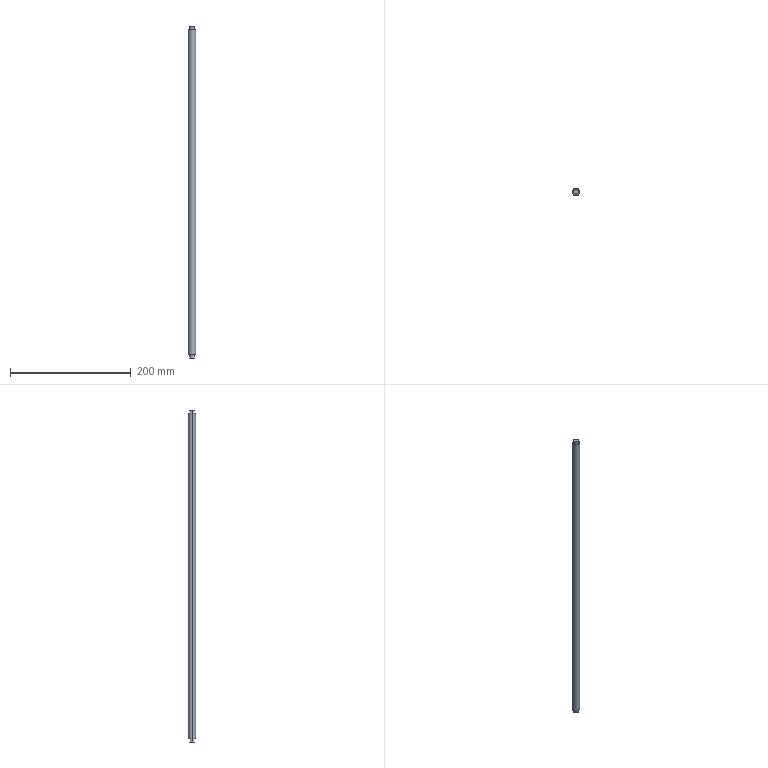Component | SolidWorks | ORTA M_L-2 | 1 solid | 10 faces | box 12 x 12 x 550 mm | volume 61575 mm3 | cylinder 6 | plane 4 | commonest cylinder face diameters 8 x4 12 x2
build123d program:
from build123d import *

# Parameters (mm, degrees)
IZIM1_R                     = 6
Y_KSEKLIK_EKSTR_ZYON1_DEPTH = 540
IZIM2_R                     = 4
Y_KSEKLIK_EKSTR_ZYON2_DEPTH = 5
Y_KSEKLIK_EKSTR_ZYON3_START = 5
IZIM3_R                     = 4
Y_KSEKLIK_EKSTR_ZYON3_DEPTH = 5


with BuildPart() as part:
    # izim1 → Y_kseklik-Ekstr_zyon1 (new body)
    with BuildSketch(Plane.XY):
        Circle(IZIM1_R)
    extrude(amount=Y_KSEKLIK_EKSTR_ZYON1_DEPTH)

    # izim2 → Y_kseklik-Ekstr_zyon2 (add)
    with BuildSketch(Plane.XY.offset(540)):
        Circle(IZIM2_R)
    extrude(amount=Y_KSEKLIK_EKSTR_ZYON2_DEPTH)

    # izim3 → Y_kseklik-Ekstr_zyon3 (add)
    with BuildSketch(Plane(origin=(0, 0, 0), x_dir=(-1, 0, 0), z_dir=(0, 0, -1)).offset(Y_KSEKLIK_EKSTR_ZYON3_START)):
        with Locations(Location((0, 0, 0), (0, 0, 180))):
            Circle(IZIM3_R)
    extrude(amount=-Y_KSEKLIK_EKSTR_ZYON3_DEPTH)


solid = part.part

# Placed as in the assembly
solid = solid.moved(Location((228.852, 24.677, -357.526), (0, 0, 0)))
STEP:
#1=COLOUR_RGB('',0.7922,0.8196,0.9333);
#2=FILL_AREA_STYLE_COLOUR('',#1);
#3=FILL_AREA_STYLE('',(#2));
#4=SURFACE_STYLE_FILL_AREA(#3);
#5=SURFACE_SIDE_STYLE('',(#4));
#6=SURFACE_STYLE_USAGE(.BOTH.,#5);
#7=PRESENTATION_STYLE_ASSIGNMENT((#6));
#8=CARTESIAN_POINT('',(8.852,0.9715,-14.273));
#9=VERTEX_POINT('',#8);
#10=CARTESIAN_POINT('',(9.167,0.9715,-14.273));
#11=VERTEX_POINT('',#10);
#12=CARTESIAN_POINT('',(9.01,0.9715,-14.273));
#13=DIRECTION('',(0.,0.,-1.));
#14=DIRECTION('',(-1.,0.,0.));
#15=AXIS2_PLACEMENT_3D('',#12,#13,#14);
#16=CIRCLE('',#15,0.1575);
#17=EDGE_CURVE('',#9,#11,#16,.T.);
#18=ORIENTED_EDGE('',*,*,#17,.F.);
#19=CARTESIAN_POINT('',(8.852,0.9715,-14.076));
#20=VERTEX_POINT('',#19);
#21=CARTESIAN_POINT('',(8.852,0.9715,-14.273));
#22=DIRECTION('',(0.,0.,1.));
#23=VECTOR('',#22,39.37);
#24=LINE('',#21,#23);
#25=EDGE_CURVE('',#9,#20,#24,.T.);
#26=ORIENTED_EDGE('',*,*,#25,.T.);
#27=CARTESIAN_POINT('',(9.167,0.9715,-14.076));
#28=VERTEX_POINT('',#27);
#29=CARTESIAN_POINT('',(9.01,0.9715,-14.076));
#30=DIRECTION('',(0.,0.,-1.));
#31=DIRECTION('',(-1.,0.,0.));
#32=AXIS2_PLACEMENT_3D('',#29,#30,#31);
#33=CIRCLE('',#32,0.1575);
#34=EDGE_CURVE('',#20,#28,#33,.T.);
#35=ORIENTED_EDGE('',*,*,#34,.T.);
#36=CARTESIAN_POINT('',(9.167,0.9715,-14.273));
#37=DIRECTION('',(0.,0.,1.));
#38=VECTOR('',#37,39.37);
#39=LINE('',#36,#38);
#40=EDGE_CURVE('',#11,#28,#39,.T.);
#41=ORIENTED_EDGE('',*,*,#40,.F.);
#42=EDGE_LOOP('',(#18,#26,#35,#41));
#43=FACE_OUTER_BOUND('',#42,.T.);
#44=CARTESIAN_POINT('',(9.01,0.9715,-14.273));
#45=DIRECTION('',(0.,0.,1.));
#46=DIRECTION('',(1.,0.,0.));
#47=AXIS2_PLACEMENT_3D('',#44,#45,#46);
#48=CYLINDRICAL_SURFACE('',#47,0.1575);
#49=ADVANCED_FACE('',(#43),#48,.T.);
#50=CARTESIAN_POINT('',(9.167,0.9715,7.381));
#51=VERTEX_POINT('',#50);
#52=CARTESIAN_POINT('',(8.852,0.9715,7.381));
#53=VERTEX_POINT('',#52);
#54=CARTESIAN_POINT('',(9.01,0.9715,7.381));
#55=DIRECTION('',(0.,0.,1.));
#56=DIRECTION('',(1.,0.,0.));
#57=AXIS2_PLACEMENT_3D('',#54,#55,#56);
#58=CIRCLE('',#57,0.1575);
#59=EDGE_CURVE('',#51,#53,#58,.T.);
#60=ORIENTED_EDGE('',*,*,#59,.F.);
#61=CARTESIAN_POINT('',(9.167,0.9715,7.184));
#62=VERTEX_POINT('',#61);
#63=CARTESIAN_POINT('',(9.167,0.9715,7.381));
#64=DIRECTION('',(0.,0.,-1.));
#65=VECTOR('',#64,39.37);
#66=LINE('',#63,#65);
#67=EDGE_CURVE('',#51,#62,#66,.T.);
#68=ORIENTED_EDGE('',*,*,#67,.T.);
#69=CARTESIAN_POINT('',(8.852,0.9715,7.184));
#70=VERTEX_POINT('',#69);
#71=CARTESIAN_POINT('',(9.01,0.9715,7.184));
#72=DIRECTION('',(0.,0.,1.));
#73=DIRECTION('',(1.,0.,0.));
#74=AXIS2_PLACEMENT_3D('',#71,#72,#73);
#75=CIRCLE('',#74,0.1575);
#76=EDGE_CURVE('',#62,#70,#75,.T.);
#77=ORIENTED_EDGE('',*,*,#76,.T.);
#78=CARTESIAN_POINT('',(8.852,0.9715,7.381));
#79=DIRECTION('',(0.,0.,-1.));
#80=VECTOR('',#79,39.37);
#81=LINE('',#78,#80);
#82=EDGE_CURVE('',#53,#70,#81,.T.);
#83=ORIENTED_EDGE('',*,*,#82,.F.);
#84=EDGE_LOOP('',(#60,#68,#77,#83));
#85=FACE_OUTER_BOUND('',#84,.T.);
#86=CARTESIAN_POINT('',(9.01,0.9715,7.381));
#87=DIRECTION('',(0.,0.,-1.));
#88=DIRECTION('',(-1.,0.,0.));
#89=AXIS2_PLACEMENT_3D('',#86,#87,#88);
#90=CYLINDRICAL_SURFACE('',#89,0.1575);
#91=ADVANCED_FACE('',(#85),#90,.T.);
#92=CARTESIAN_POINT('',(9.246,0.9715,7.184));
#93=VERTEX_POINT('',#92);
#94=CARTESIAN_POINT('',(8.774,0.9715,7.184));
#95=VERTEX_POINT('',#94);
#96=CARTESIAN_POINT('',(9.01,0.9715,7.184));
#97=DIRECTION('',(0.,0.,1.));
#98=DIRECTION('',(1.,0.,0.));
#99=AXIS2_PLACEMENT_3D('',#96,#97,#98);
#100=CIRCLE('',#99,0.2362);
#101=EDGE_CURVE('',#93,#95,#100,.T.);
#102=ORIENTED_EDGE('',*,*,#101,.F.);
#103=CARTESIAN_POINT('',(9.246,0.9715,-14.076));
#104=VERTEX_POINT('',#103);
#105=CARTESIAN_POINT('',(9.246,0.9715,7.184));
#106=DIRECTION('',(0.,0.,-1.));
#107=VECTOR('',#106,39.37);
#108=LINE('',#105,#107);
#109=EDGE_CURVE('',#93,#104,#108,.T.);
#110=ORIENTED_EDGE('',*,*,#109,.T.);
#111=CARTESIAN_POINT('',(8.774,0.9715,-14.076));
#112=VERTEX_POINT('',#111);
#113=CARTESIAN_POINT('',(9.01,0.9715,-14.076));
#114=DIRECTION('',(0.,0.,1.));
#115=DIRECTION('',(1.,0.,0.));
#116=AXIS2_PLACEMENT_3D('',#113,#114,#115);
#117=CIRCLE('',#116,0.2362);
#118=EDGE_CURVE('',#104,#112,#117,.T.);
#119=ORIENTED_EDGE('',*,*,#118,.T.);
#120=CARTESIAN_POINT('',(8.774,0.9715,7.184));
#121=DIRECTION('',(0.,0.,-1.));
#122=VECTOR('',#121,39.37);
#123=LINE('',#120,#122);
#124=EDGE_CURVE('',#95,#112,#123,.T.);
#125=ORIENTED_EDGE('',*,*,#124,.F.);
#126=EDGE_LOOP('',(#102,#110,#119,#125));
#127=FACE_OUTER_BOUND('',#126,.T.);
#128=CARTESIAN_POINT('',(9.01,0.9715,7.184));
#129=DIRECTION('',(0.,0.,-1.));
#130=DIRECTION('',(-1.,0.,0.));
#131=AXIS2_PLACEMENT_3D('',#128,#129,#130);
#132=CYLINDRICAL_SURFACE('',#131,0.2362);
#133=ADVANCED_FACE('',(#127),#132,.T.);
#134=ORIENTED_EDGE('',*,*,#109,.F.);
#135=CARTESIAN_POINT('',(9.01,0.9715,7.184));
#136=DIRECTION('',(0.,0.,1.));
#137=DIRECTION('',(1.,0.,0.));
#138=AXIS2_PLACEMENT_3D('',#135,#136,#137);
#139=CIRCLE('',#138,0.2362);
#140=EDGE_CURVE('',#95,#93,#139,.T.);
#141=ORIENTED_EDGE('',*,*,#140,.F.);
#142=ORIENTED_EDGE('',*,*,#124,.T.);
#143=CARTESIAN_POINT('',(9.01,0.9715,-14.076));
#144=DIRECTION('',(0.,0.,1.));
#145=DIRECTION('',(1.,0.,0.));
#146=AXIS2_PLACEMENT_3D('',#143,#144,#145);
#147=CIRCLE('',#146,0.2362);
#148=EDGE_CURVE('',#112,#104,#147,.T.);
#149=ORIENTED_EDGE('',*,*,#148,.T.);
#150=EDGE_LOOP('',(#134,#141,#142,#149));
#151=FACE_OUTER_BOUND('',#150,.T.);
#152=CARTESIAN_POINT('',(9.01,0.9715,7.184));
#153=DIRECTION('',(0.,0.,-1.));
#154=DIRECTION('',(-1.,0.,0.));
#155=AXIS2_PLACEMENT_3D('',#152,#153,#154);
#156=CYLINDRICAL_SURFACE('',#155,0.2362);
#157=ADVANCED_FACE('',(#151),#156,.T.);
#158=CARTESIAN_POINT('',(9.01,0.9715,7.184));
#159=DIRECTION('',(0.,0.,1.));
#160=DIRECTION('',(1.,0.,0.));
#161=AXIS2_PLACEMENT_3D('',#158,#159,#160);
#162=CIRCLE('',#161,0.1575);
#163=EDGE_CURVE('',#70,#62,#162,.T.);
#164=ORIENTED_EDGE('',*,*,#163,.F.);
#165=ORIENTED_EDGE('',*,*,#76,.F.);
#166=EDGE_LOOP('',(#164,#165));
#167=FACE_BOUND('',#166,.T.);
#168=ORIENTED_EDGE('',*,*,#140,.T.);
#169=ORIENTED_EDGE('',*,*,#101,.T.);
#170=EDGE_LOOP('',(#168,#169));
#171=FACE_OUTER_BOUND('',#170,.T.);
#172=CARTESIAN_POINT('',(9.01,0.9715,7.184));
#173=DIRECTION('',(0.,0.,1.));
#174=DIRECTION('',(1.,0.,0.));
#175=AXIS2_PLACEMENT_3D('',#172,#173,#174);
#176=PLANE('',#175);
#177=ADVANCED_FACE('',(#167,#171),#176,.T.);
#178=CARTESIAN_POINT('',(9.01,0.9715,-14.076));
#179=DIRECTION('',(0.,0.,-1.));
#180=DIRECTION('',(-1.,0.,0.));
#181=AXIS2_PLACEMENT_3D('',#178,#179,#180);
#182=CIRCLE('',#181,0.1575);
#183=EDGE_CURVE('',#28,#20,#182,.T.);
#184=ORIENTED_EDGE('',*,*,#183,.F.);
#185=ORIENTED_EDGE('',*,*,#34,.F.);
#186=EDGE_LOOP('',(#184,#185));
#187=FACE_BOUND('',#186,.T.);
#188=ORIENTED_EDGE('',*,*,#148,.F.);
#189=ORIENTED_EDGE('',*,*,#118,.F.);
#190=EDGE_LOOP('',(#188,#189));
#191=FACE_OUTER_BOUND('',#190,.T.);
#192=CARTESIAN_POINT('',(9.01,0.9715,-14.076));
#193=DIRECTION('',(0.,0.,1.));
#194=DIRECTION('',(1.,0.,0.));
#195=AXIS2_PLACEMENT_3D('',#192,#193,#194);
#196=PLANE('',#195);
#197=ADVANCED_FACE('',(#187,#191),#196,.F.);
#198=ORIENTED_EDGE('',*,*,#67,.F.);
#199=CARTESIAN_POINT('',(9.01,0.9715,7.381));
#200=DIRECTION('',(0.,0.,1.));
#201=DIRECTION('',(1.,0.,0.));
#202=AXIS2_PLACEMENT_3D('',#199,#200,#201);
#203=CIRCLE('',#202,0.1575);
#204=EDGE_CURVE('',#53,#51,#203,.T.);
#205=ORIENTED_EDGE('',*,*,#204,.F.);
#206=ORIENTED_EDGE('',*,*,#82,.T.);
#207=ORIENTED_EDGE('',*,*,#163,.T.);
#208=EDGE_LOOP('',(#198,#205,#206,#207));
#209=FACE_OUTER_BOUND('',#208,.T.);
#210=CARTESIAN_POINT('',(9.01,0.9715,7.381));
#211=DIRECTION('',(0.,0.,-1.));
#212=DIRECTION('',(-1.,0.,0.));
#213=AXIS2_PLACEMENT_3D('',#210,#211,#212);
#214=CYLINDRICAL_SURFACE('',#213,0.1575);
#215=ADVANCED_FACE('',(#209),#214,.T.);
#216=ORIENTED_EDGE('',*,*,#204,.T.);
#217=ORIENTED_EDGE('',*,*,#59,.T.);
#218=EDGE_LOOP('',(#216,#217));
#219=FACE_OUTER_BOUND('',#218,.T.);
#220=CARTESIAN_POINT('',(9.01,0.9715,7.381));
#221=DIRECTION('',(0.,0.,1.));
#222=DIRECTION('',(1.,0.,0.));
#223=AXIS2_PLACEMENT_3D('',#220,#221,#222);
#224=PLANE('',#223);
#225=ADVANCED_FACE('',(#219),#224,.T.);
#226=ORIENTED_EDGE('',*,*,#25,.F.);
#227=CARTESIAN_POINT('',(9.01,0.9715,-14.273));
#228=DIRECTION('',(0.,0.,-1.));
#229=DIRECTION('',(-1.,0.,0.));
#230=AXIS2_PLACEMENT_3D('',#227,#228,#229);
#231=CIRCLE('',#230,0.1575);
#232=EDGE_CURVE('',#11,#9,#231,.T.);
#233=ORIENTED_EDGE('',*,*,#232,.F.);
#234=ORIENTED_EDGE('',*,*,#40,.T.);
#235=ORIENTED_EDGE('',*,*,#183,.T.);
#236=EDGE_LOOP('',(#226,#233,#234,#235));
#237=FACE_OUTER_BOUND('',#236,.T.);
#238=CARTESIAN_POINT('',(9.01,0.9715,-14.273));
#239=DIRECTION('',(0.,0.,1.));
#240=DIRECTION('',(1.,0.,0.));
#241=AXIS2_PLACEMENT_3D('',#238,#239,#240);
#242=CYLINDRICAL_SURFACE('',#241,0.1575);
#243=ADVANCED_FACE('',(#237),#242,.T.);
#244=ORIENTED_EDGE('',*,*,#232,.T.);
#245=ORIENTED_EDGE('',*,*,#17,.T.);
#246=EDGE_LOOP('',(#244,#245));
#247=FACE_OUTER_BOUND('',#246,.T.);
#248=CARTESIAN_POINT('',(9.01,0.9715,-14.273));
#249=DIRECTION('',(0.,0.,-1.));
#250=DIRECTION('',(-1.,0.,0.));
#251=AXIS2_PLACEMENT_3D('',#248,#249,#250);
#252=PLANE('',#251);
#253=ADVANCED_FACE('',(#247),#252,.T.);
#254=CLOSED_SHELL('',(#49,#91,#133,#157,#177,#197,#215,#225,#243,#253));
#255=MANIFOLD_SOLID_BREP('',#254);
#256=STYLED_ITEM('',(#7),#255);
#257=(LENGTH_UNIT()NAMED_UNIT(*)SI_UNIT($,.METRE.));
#258=LENGTH_MEASURE_WITH_UNIT(LENGTH_MEASURE(0.0254),#257);
#259=DIMENSIONAL_EXPONENTS(1.,0.,0.,0.,0.,0.,0.);
#260=(CONVERSION_BASED_UNIT('',#258)LENGTH_UNIT()NAMED_UNIT(#259));
#261=UNCERTAINTY_MEASURE_WITH_UNIT(LENGTH_MEASURE(0.00001),#260,'','');
#262=(NAMED_UNIT(*)PLANE_ANGLE_UNIT()SI_UNIT($,.RADIAN.));
#263=(NAMED_UNIT(*)SI_UNIT($,.STERADIAN.)SOLID_ANGLE_UNIT());
#264=(GEOMETRIC_REPRESENTATION_CONTEXT(3)GLOBAL_UNCERTAINTY_ASSIGNED_CONTEXT((#261))GLOBAL_UNIT_ASSIGNED_CONTEXT((#260,#262,#263))REPRESENTATION_CONTEXT('',''));
#265=MECHANICAL_DESIGN_GEOMETRIC_PRESENTATION_REPRESENTATION('',(#256),#264);
#266=PRESENTATION_LAYER_ASSIGNMENT('','',(#256));
#267=CARTESIAN_POINT('',(0.,0.,0.));
#268=DIRECTION('',(0.,0.,1.));
#269=DIRECTION('',(1.,0.,0.));
#270=AXIS2_PLACEMENT_3D('',#267,#268,#269);
#271=(LENGTH_UNIT()NAMED_UNIT(*)SI_UNIT($,.METRE.));
#272=LENGTH_MEASURE_WITH_UNIT(LENGTH_MEASURE(0.0254),#271);
#273=DIMENSIONAL_EXPONENTS(1.,0.,0.,0.,0.,0.,0.);
#274=(CONVERSION_BASED_UNIT('',#272)LENGTH_UNIT()NAMED_UNIT(#273));
#275=UNCERTAINTY_MEASURE_WITH_UNIT(LENGTH_MEASURE(0.00001),#274,'','');
#276=(NAMED_UNIT(*)PLANE_ANGLE_UNIT()SI_UNIT($,.RADIAN.));
#277=(NAMED_UNIT(*)SI_UNIT($,.STERADIAN.)SOLID_ANGLE_UNIT());
#278=(GEOMETRIC_REPRESENTATION_CONTEXT(3)GLOBAL_UNCERTAINTY_ASSIGNED_CONTEXT((#275))GLOBAL_UNIT_ASSIGNED_CONTEXT((#274,#276,#277))REPRESENTATION_CONTEXT('',''));
#279=ADVANCED_BREP_SHAPE_REPRESENTATION('',(#255,#270),#278);